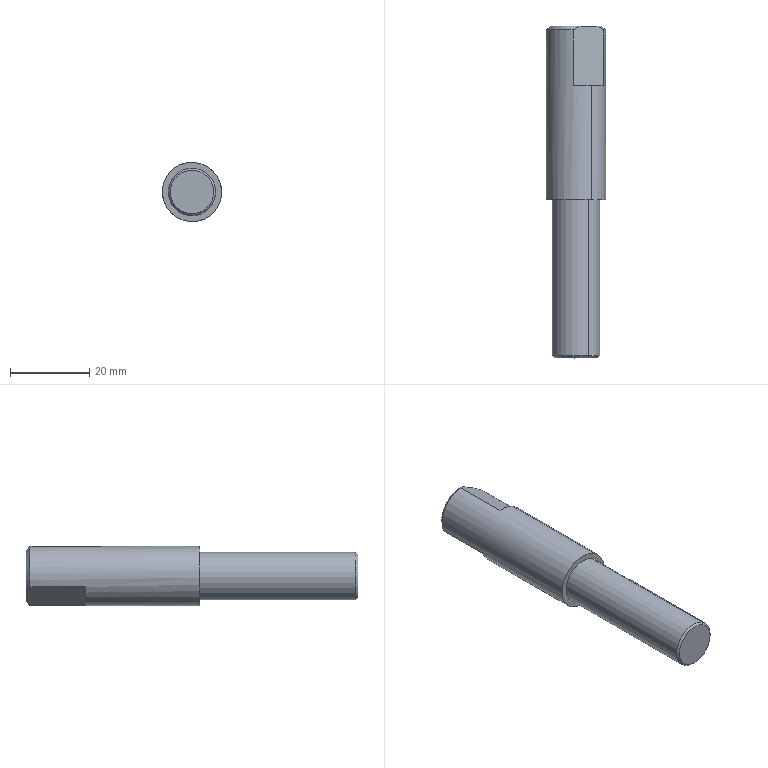Component | SolidWorks | GbgbLowerMagnetPushRodF8-1 | 1 solid | 19 faces | box 15 x 84 x 15 mm | volume 11648 mm3 | plane 7 | cone 6 | cylinder 6 | commonest cylinder face diameters 6 x2 12 x2 15 x2
build123d program:
from build123d import *

# Parameters (mm, degrees)
M6_TAPPED_HOLE1_D     = 6
M6_TAPPED_HOLE1_DEPTH = 12
M6_TAPPED_HOLE1_TIP   = 1.803
SKETCH4_OUTSIDE_W     = 34.328
SKETCH4_OUTSIDE_H     = 34.328
SKETCH4_OUTSIDE_W_2   = 23.531
SKETCH4_OUTSIDE_H_2   = 12
CUT_EXTRUDE1_DEPTH    = 15
CHAMFER2_SIZE         = 0.5
CHAMFER3_SIZE         = 1


with BuildPart() as part:
    # Sketch1 → Revolve1 (revolve)
    with BuildSketch(Plane.XY, mode=Mode.PRIVATE) as revolve1_sk:
        Polygon((0, 40), (-6, 40), (-6, 0), (-7.5, 0), (-7.5, -44), (0, -44), align=None)
    revolve(revolve1_sk.sketch.rotate(Axis((0, 59.694, 0), (0, -1, 0)), 270), axis=Axis((0, 59.694, 0), (0, -1, 0)))

    # M6 Tapped Hole1
    with Locations(Plane(origin=(0, -44, 0), x_dir=(-1, 0, 0), z_dir=(0, -1, 0))):
        with Locations((0, 0)):
            Hole(M6_TAPPED_HOLE1_D / 2, depth=M6_TAPPED_HOLE1_DEPTH)
            with Locations((0, 0, -(M6_TAPPED_HOLE1_DEPTH + M6_TAPPED_HOLE1_TIP / 2))):  # 118° drill point
                Cone(0, M6_TAPPED_HOLE1_D / 2, M6_TAPPED_HOLE1_TIP, mode=Mode.SUBTRACT)

    # Sketch4 outside → Cut-Extrude1 (cut)
    with BuildSketch(Plane.XZ.offset(44)):
        Rectangle(SKETCH4_OUTSIDE_W, SKETCH4_OUTSIDE_H)
        Rectangle(SKETCH4_OUTSIDE_W_2, SKETCH4_OUTSIDE_H_2, mode=Mode.SUBTRACT)
    extrude(amount=-CUT_EXTRUDE1_DEPTH, mode=Mode.SUBTRACT)

    # Chamfer2
    chamfer2_edges = [part.edges().sort_by_distance(p)[0] for p in [
        (0, 40, -6),
    ]]
    chamfer(chamfer2_edges, length=CHAMFER2_SIZE)

    # Chamfer3
    chamfer3_edges = [part.edges().sort_by_distance(p)[0] for p in [
        (-7.5, -44, 0),
        (7.5, -44, 0),
    ]]
    chamfer(chamfer3_edges, length=CHAMFER3_SIZE)


solid = part.part

# Placed as in the assembly
solid = solid.moved(Location((80.446, 428.93, 430.232), (0, 31.476, -180)))
STEP:
#1=CARTESIAN_POINT('',(3.054,15.312,16.754));
#2=VERTEX_POINT('',#1);
#3=CARTESIAN_POINT('',(3.28,15.312,17.123));
#4=VERTEX_POINT('',#3);
#5=CARTESIAN_POINT('',(3.167,15.312,16.938));
#6=DIRECTION('',(-0.,-1.,-0.));
#7=DIRECTION('',(-0.5221,0.,-0.8529));
#8=AXIS2_PLACEMENT_3D('',#5,#6,#7);
#9=CIRCLE('',#8,0.2165);
#10=EDGE_CURVE('',#2,#4,#9,.T.);
#11=ORIENTED_EDGE('',*,*,#10,.F.);
#12=CARTESIAN_POINT('',(3.044,15.332,16.737));
#13=VERTEX_POINT('',#12);
#14=CARTESIAN_POINT('',(3.054,15.312,16.754));
#15=DIRECTION('',(-0.3692,0.7071,-0.6031));
#16=VECTOR('',#15,39.37);
#17=LINE('',#14,#16);
#18=EDGE_CURVE('',#2,#13,#17,.T.);
#19=ORIENTED_EDGE('',*,*,#18,.T.);
#20=CARTESIAN_POINT('',(3.291,15.332,17.14));
#21=VERTEX_POINT('',#20);
#22=CARTESIAN_POINT('',(3.167,15.332,16.938));
#23=DIRECTION('',(0.,1.,0.));
#24=DIRECTION('',(-0.5221,0.,-0.8529));
#25=AXIS2_PLACEMENT_3D('',#22,#23,#24);
#26=CIRCLE('',#25,0.2362);
#27=EDGE_CURVE('',#21,#13,#26,.T.);
#28=ORIENTED_EDGE('',*,*,#27,.F.);
#29=CARTESIAN_POINT('',(3.28,15.312,17.123));
#30=DIRECTION('',(0.3692,0.7071,0.6031));
#31=VECTOR('',#30,39.37);
#32=LINE('',#29,#31);
#33=EDGE_CURVE('',#4,#21,#32,.T.);
#34=ORIENTED_EDGE('',*,*,#33,.F.);
#35=EDGE_LOOP('',(#11,#19,#28,#34));
#36=FACE_OUTER_BOUND('',#35,.T.);
#37=CARTESIAN_POINT('',(3.167,15.312,16.938));
#38=DIRECTION('',(0.,1.,0.));
#39=DIRECTION('',(0.5221,0.,0.8529));
#40=AXIS2_PLACEMENT_3D('',#37,#38,#39);
#41=CONICAL_SURFACE('',#40,0.2165,0.7854);
#42=ADVANCED_FACE('',(#36),#41,.T.);
#43=CARTESIAN_POINT('',(3.106,18.147,16.838));
#44=VERTEX_POINT('',#43);
#45=CARTESIAN_POINT('',(3.229,18.147,17.039));
#46=VERTEX_POINT('',#45);
#47=CARTESIAN_POINT('',(3.167,18.147,16.938));
#48=DIRECTION('',(0.,1.,0.));
#49=DIRECTION('',(0.5221,0.,0.8529));
#50=AXIS2_PLACEMENT_3D('',#47,#48,#49);
#51=CIRCLE('',#50,0.1181);
#52=EDGE_CURVE('',#44,#46,#51,.T.);
#53=ORIENTED_EDGE('',*,*,#52,.F.);
#54=CARTESIAN_POINT('',(3.106,18.619,16.838));
#55=VERTEX_POINT('',#54);
#56=CARTESIAN_POINT('',(3.106,18.619,16.838));
#57=DIRECTION('',(0.,1.,0.));
#58=VECTOR('',#57,39.37);
#59=LINE('',#56,#58);
#60=EDGE_CURVE('',#44,#55,#59,.T.);
#61=ORIENTED_EDGE('',*,*,#60,.T.);
#62=CARTESIAN_POINT('',(3.229,18.619,17.039));
#63=VERTEX_POINT('',#62);
#64=CARTESIAN_POINT('',(3.167,18.619,16.938));
#65=DIRECTION('',(0.,1.,0.));
#66=DIRECTION('',(0.5221,0.,0.8529));
#67=AXIS2_PLACEMENT_3D('',#64,#65,#66);
#68=CIRCLE('',#67,0.1181);
#69=EDGE_CURVE('',#55,#63,#68,.T.);
#70=ORIENTED_EDGE('',*,*,#69,.T.);
#71=CARTESIAN_POINT('',(3.229,18.619,17.039));
#72=DIRECTION('',(0.,1.,0.));
#73=VECTOR('',#72,39.37);
#74=LINE('',#71,#73);
#75=EDGE_CURVE('',#46,#63,#74,.T.);
#76=ORIENTED_EDGE('',*,*,#75,.F.);
#77=EDGE_LOOP('',(#53,#61,#70,#76));
#78=FACE_OUTER_BOUND('',#77,.T.);
#79=CARTESIAN_POINT('',(3.167,18.619,16.938));
#80=DIRECTION('',(0.,1.,0.));
#81=DIRECTION('',(0.5221,0.,0.8529));
#82=AXIS2_PLACEMENT_3D('',#79,#80,#81);
#83=CYLINDRICAL_SURFACE('',#82,0.1181);
#84=ADVANCED_FACE('',(#78),#83,.F.);
#85=CARTESIAN_POINT('',(3.167,18.076,16.938));
#86=VERTEX_POINT('',#85);
#87=CARTESIAN_POINT('',(3.229,18.147,17.039));
#88=DIRECTION('',(0.4476,0.515,0.731));
#89=VECTOR('',#88,39.37);
#90=LINE('',#87,#89);
#91=EDGE_CURVE('',#86,#46,#90,.T.);
#92=ORIENTED_EDGE('',*,*,#91,.F.);
#93=CARTESIAN_POINT('',(3.106,18.147,16.838));
#94=DIRECTION('',(-0.4476,0.515,-0.731));
#95=VECTOR('',#94,39.37);
#96=LINE('',#93,#95);
#97=EDGE_CURVE('',#86,#44,#96,.T.);
#98=ORIENTED_EDGE('',*,*,#97,.T.);
#99=ORIENTED_EDGE('',*,*,#52,.T.);
#100=EDGE_LOOP('',(#92,#98,#99));
#101=FACE_OUTER_BOUND('',#100,.T.);
#102=CARTESIAN_POINT('',(3.167,18.147,16.938));
#103=DIRECTION('',(0.,1.,0.));
#104=DIRECTION('',(0.5221,0.,0.8529));
#105=AXIS2_PLACEMENT_3D('',#102,#103,#104);
#106=CONICAL_SURFACE('',#105,0.1181,1.03);
#107=ADVANCED_FACE('',(#101),#106,.F.);
#108=CARTESIAN_POINT('',(3.044,16.887,16.737));
#109=VERTEX_POINT('',#108);
#110=CARTESIAN_POINT('',(3.291,16.887,17.14));
#111=VERTEX_POINT('',#110);
#112=CARTESIAN_POINT('',(3.167,16.887,16.938));
#113=DIRECTION('',(-0.,-1.,-0.));
#114=DIRECTION('',(-0.5221,0.,-0.8529));
#115=AXIS2_PLACEMENT_3D('',#112,#113,#114);
#116=CIRCLE('',#115,0.2362);
#117=EDGE_CURVE('',#109,#111,#116,.T.);
#118=ORIENTED_EDGE('',*,*,#117,.T.);
#119=CARTESIAN_POINT('',(3.291,14.537,17.14));
#120=DIRECTION('',(-0.,-1.,-0.));
#121=VECTOR('',#120,39.37);
#122=LINE('',#119,#121);
#123=EDGE_CURVE('',#111,#21,#122,.T.);
#124=ORIENTED_EDGE('',*,*,#123,.T.);
#125=ORIENTED_EDGE('',*,*,#27,.T.);
#126=CARTESIAN_POINT('',(3.044,14.537,16.737));
#127=DIRECTION('',(-0.,-1.,-0.));
#128=VECTOR('',#127,39.37);
#129=LINE('',#126,#128);
#130=EDGE_CURVE('',#109,#13,#129,.T.);
#131=ORIENTED_EDGE('',*,*,#130,.F.);
#132=EDGE_LOOP('',(#118,#124,#125,#131));
#133=FACE_OUTER_BOUND('',#132,.T.);
#134=CARTESIAN_POINT('',(3.167,14.537,16.938));
#135=DIRECTION('',(-0.,-1.,-0.));
#136=DIRECTION('',(-0.5221,0.,-0.8529));
#137=AXIS2_PLACEMENT_3D('',#134,#135,#136);
#138=CYLINDRICAL_SURFACE('',#137,0.2362);
#139=ADVANCED_FACE('',(#133),#138,.T.);
#140=CARTESIAN_POINT('',(3.442,18.029,17.047));
#141=VERTEX_POINT('',#140);
#142=CARTESIAN_POINT('',(3.321,18.029,17.19));
#143=VERTEX_POINT('',#142);
#144=CARTESIAN_POINT('',(3.167,18.029,16.938));
#145=DIRECTION('',(-0.,-1.,-0.));
#146=DIRECTION('',(0.5221,0.,0.8529));
#147=AXIS2_PLACEMENT_3D('',#144,#145,#146);
#148=CIRCLE('',#147,0.2953);
#149=EDGE_CURVE('',#141,#143,#148,.T.);
#150=ORIENTED_EDGE('',*,*,#149,.T.);
#151=CARTESIAN_POINT('',(3.321,16.887,17.19));
#152=VERTEX_POINT('',#151);
#153=CARTESIAN_POINT('',(3.321,14.537,17.19));
#154=DIRECTION('',(-0.,-1.,-0.));
#155=VECTOR('',#154,39.37);
#156=LINE('',#153,#155);
#157=EDGE_CURVE('',#143,#152,#156,.T.);
#158=ORIENTED_EDGE('',*,*,#157,.T.);
#159=CARTESIAN_POINT('',(3.013,16.887,16.686));
#160=VERTEX_POINT('',#159);
#161=CARTESIAN_POINT('',(3.167,16.887,16.938));
#162=DIRECTION('',(-0.,-1.,-0.));
#163=DIRECTION('',(-0.5221,0.,-0.8529));
#164=AXIS2_PLACEMENT_3D('',#161,#162,#163);
#165=CIRCLE('',#164,0.2953);
#166=EDGE_CURVE('',#160,#152,#165,.T.);
#167=ORIENTED_EDGE('',*,*,#166,.F.);
#168=CARTESIAN_POINT('',(3.013,18.029,16.686));
#169=VERTEX_POINT('',#168);
#170=CARTESIAN_POINT('',(3.013,14.537,16.686));
#171=DIRECTION('',(-0.,-1.,-0.));
#172=VECTOR('',#171,39.37);
#173=LINE('',#170,#172);
#174=EDGE_CURVE('',#169,#160,#173,.T.);
#175=ORIENTED_EDGE('',*,*,#174,.F.);
#176=CARTESIAN_POINT('',(3.195,18.029,16.644));
#177=VERTEX_POINT('',#176);
#178=CARTESIAN_POINT('',(3.167,18.029,16.938));
#179=DIRECTION('',(-0.,-1.,-0.));
#180=DIRECTION('',(0.5221,0.,0.8529));
#181=AXIS2_PLACEMENT_3D('',#178,#179,#180);
#182=CIRCLE('',#181,0.2953);
#183=EDGE_CURVE('',#169,#177,#182,.T.);
#184=ORIENTED_EDGE('',*,*,#183,.T.);
#185=CARTESIAN_POINT('',(3.195,18.58,16.644));
#186=VERTEX_POINT('',#185);
#187=CARTESIAN_POINT('',(3.195,14.537,16.644));
#188=DIRECTION('',(0.,1.,0.));
#189=VECTOR('',#188,39.37);
#190=LINE('',#187,#189);
#191=EDGE_CURVE('',#177,#186,#190,.T.);
#192=ORIENTED_EDGE('',*,*,#191,.T.);
#193=CARTESIAN_POINT('',(3.442,18.58,17.047));
#194=VERTEX_POINT('',#193);
#195=CARTESIAN_POINT('',(3.167,18.58,16.938));
#196=DIRECTION('',(-0.,-1.,-0.));
#197=DIRECTION('',(0.5221,0.,0.8529));
#198=AXIS2_PLACEMENT_3D('',#195,#196,#197);
#199=CIRCLE('',#198,0.2953);
#200=EDGE_CURVE('',#186,#194,#199,.T.);
#201=ORIENTED_EDGE('',*,*,#200,.T.);
#202=CARTESIAN_POINT('',(3.442,14.537,17.047));
#203=DIRECTION('',(-0.,-1.,-0.));
#204=VECTOR('',#203,39.37);
#205=LINE('',#202,#204);
#206=EDGE_CURVE('',#194,#141,#205,.T.);
#207=ORIENTED_EDGE('',*,*,#206,.T.);
#208=EDGE_LOOP('',(#150,#158,#167,#175,#184,#192,#201,#207));
#209=FACE_OUTER_BOUND('',#208,.T.);
#210=CARTESIAN_POINT('',(3.167,14.537,16.938));
#211=DIRECTION('',(-0.,-1.,-0.));
#212=DIRECTION('',(-0.5221,0.,-0.8529));
#213=AXIS2_PLACEMENT_3D('',#210,#211,#212);
#214=CYLINDRICAL_SURFACE('',#213,0.2953);
#215=ADVANCED_FACE('',(#209),#214,.T.);
#216=ORIENTED_EDGE('',*,*,#157,.F.);
#217=CARTESIAN_POINT('',(3.139,18.029,17.232));
#218=VERTEX_POINT('',#217);
#219=CARTESIAN_POINT('',(3.167,18.029,16.938));
#220=DIRECTION('',(-0.,-1.,-0.));
#221=DIRECTION('',(0.5221,0.,0.8529));
#222=AXIS2_PLACEMENT_3D('',#219,#220,#221);
#223=CIRCLE('',#222,0.2953);
#224=EDGE_CURVE('',#143,#218,#223,.T.);
#225=ORIENTED_EDGE('',*,*,#224,.T.);
#226=CARTESIAN_POINT('',(3.139,18.58,17.232));
#227=VERTEX_POINT('',#226);
#228=CARTESIAN_POINT('',(3.139,14.537,17.232));
#229=DIRECTION('',(0.,1.,0.));
#230=VECTOR('',#229,39.37);
#231=LINE('',#228,#230);
#232=EDGE_CURVE('',#218,#227,#231,.T.);
#233=ORIENTED_EDGE('',*,*,#232,.T.);
#234=CARTESIAN_POINT('',(2.893,18.58,16.829));
#235=VERTEX_POINT('',#234);
#236=CARTESIAN_POINT('',(3.167,18.58,16.938));
#237=DIRECTION('',(-0.,-1.,-0.));
#238=DIRECTION('',(0.5221,0.,0.8529));
#239=AXIS2_PLACEMENT_3D('',#236,#237,#238);
#240=CIRCLE('',#239,0.2953);
#241=EDGE_CURVE('',#227,#235,#240,.T.);
#242=ORIENTED_EDGE('',*,*,#241,.T.);
#243=CARTESIAN_POINT('',(2.893,18.029,16.829));
#244=VERTEX_POINT('',#243);
#245=CARTESIAN_POINT('',(2.893,14.537,16.829));
#246=DIRECTION('',(-0.,-1.,-0.));
#247=VECTOR('',#246,39.37);
#248=LINE('',#245,#247);
#249=EDGE_CURVE('',#235,#244,#248,.T.);
#250=ORIENTED_EDGE('',*,*,#249,.T.);
#251=CARTESIAN_POINT('',(3.167,18.029,16.938));
#252=DIRECTION('',(-0.,-1.,-0.));
#253=DIRECTION('',(0.5221,0.,0.8529));
#254=AXIS2_PLACEMENT_3D('',#251,#252,#253);
#255=CIRCLE('',#254,0.2953);
#256=EDGE_CURVE('',#244,#169,#255,.T.);
#257=ORIENTED_EDGE('',*,*,#256,.T.);
#258=ORIENTED_EDGE('',*,*,#174,.T.);
#259=CARTESIAN_POINT('',(3.167,16.887,16.938));
#260=DIRECTION('',(-0.,-1.,-0.));
#261=DIRECTION('',(-0.5221,0.,-0.8529));
#262=AXIS2_PLACEMENT_3D('',#259,#260,#261);
#263=CIRCLE('',#262,0.2953);
#264=EDGE_CURVE('',#152,#160,#263,.T.);
#265=ORIENTED_EDGE('',*,*,#264,.F.);
#266=EDGE_LOOP('',(#216,#225,#233,#242,#250,#257,#258,#265));
#267=FACE_OUTER_BOUND('',#266,.T.);
#268=CARTESIAN_POINT('',(3.167,14.537,16.938));
#269=DIRECTION('',(-0.,-1.,-0.));
#270=DIRECTION('',(-0.5221,0.,-0.8529));
#271=AXIS2_PLACEMENT_3D('',#268,#269,#270);
#272=CYLINDRICAL_SURFACE('',#271,0.2953);
#273=ADVANCED_FACE('',(#267),#272,.T.);
#274=CARTESIAN_POINT('',(3.167,18.619,16.938));
#275=DIRECTION('',(0.,1.,0.));
#276=DIRECTION('',(0.5221,0.,0.8529));
#277=AXIS2_PLACEMENT_3D('',#274,#275,#276);
#278=CIRCLE('',#277,0.1181);
#279=EDGE_CURVE('',#63,#55,#278,.T.);
#280=ORIENTED_EDGE('',*,*,#279,.F.);
#281=ORIENTED_EDGE('',*,*,#69,.F.);
#282=EDGE_LOOP('',(#280,#281));
#283=FACE_BOUND('',#282,.T.);
#284=CARTESIAN_POINT('',(3.207,18.619,17.191));
#285=VERTEX_POINT('',#284);
#286=CARTESIAN_POINT('',(3.374,18.619,17.088));
#287=VERTEX_POINT('',#286);
#288=CARTESIAN_POINT('',(3.039,18.619,17.294));
#289=DIRECTION('',(0.8529,-0.,-0.5221));
#290=VECTOR('',#289,39.37);
#291=LINE('',#288,#290);
#292=EDGE_CURVE('',#285,#287,#291,.T.);
#293=ORIENTED_EDGE('',*,*,#292,.T.);
#294=CARTESIAN_POINT('',(3.128,18.619,16.685));
#295=VERTEX_POINT('',#294);
#296=CARTESIAN_POINT('',(3.167,18.619,16.938));
#297=DIRECTION('',(0.,1.,0.));
#298=DIRECTION('',(0.5221,0.,0.8529));
#299=AXIS2_PLACEMENT_3D('',#296,#297,#298);
#300=CIRCLE('',#299,0.2559);
#301=EDGE_CURVE('',#287,#295,#300,.T.);
#302=ORIENTED_EDGE('',*,*,#301,.T.);
#303=CARTESIAN_POINT('',(2.96,18.619,16.788));
#304=VERTEX_POINT('',#303);
#305=CARTESIAN_POINT('',(2.792,18.619,16.891));
#306=DIRECTION('',(-0.8529,0.,0.5221));
#307=VECTOR('',#306,39.37);
#308=LINE('',#305,#307);
#309=EDGE_CURVE('',#295,#304,#308,.T.);
#310=ORIENTED_EDGE('',*,*,#309,.T.);
#311=CARTESIAN_POINT('',(3.167,18.619,16.938));
#312=DIRECTION('',(0.,1.,0.));
#313=DIRECTION('',(0.5221,0.,0.8529));
#314=AXIS2_PLACEMENT_3D('',#311,#312,#313);
#315=CIRCLE('',#314,0.2559);
#316=EDGE_CURVE('',#304,#285,#315,.T.);
#317=ORIENTED_EDGE('',*,*,#316,.T.);
#318=EDGE_LOOP('',(#293,#302,#310,#317));
#319=FACE_OUTER_BOUND('',#318,.T.);
#320=CARTESIAN_POINT('',(2.915,18.619,17.092));
#321=DIRECTION('',(0.,1.,0.));
#322=DIRECTION('',(0.5221,-0.,0.8529));
#323=AXIS2_PLACEMENT_3D('',#320,#321,#322);
#324=PLANE('',#323);
#325=ADVANCED_FACE('',(#283,#319),#324,.T.);
#326=CARTESIAN_POINT('',(3.167,15.312,16.938));
#327=DIRECTION('',(-0.,-1.,-0.));
#328=DIRECTION('',(-0.5221,0.,-0.8529));
#329=AXIS2_PLACEMENT_3D('',#326,#327,#328);
#330=CIRCLE('',#329,0.2165);
#331=EDGE_CURVE('',#4,#2,#330,.T.);
#332=ORIENTED_EDGE('',*,*,#331,.T.);
#333=ORIENTED_EDGE('',*,*,#10,.T.);
#334=EDGE_LOOP('',(#332,#333));
#335=FACE_OUTER_BOUND('',#334,.T.);
#336=CARTESIAN_POINT('',(3.167,15.312,16.938));
#337=DIRECTION('',(-0.,-1.,-0.));
#338=DIRECTION('',(-0.5221,0.,-0.8529));
#339=AXIS2_PLACEMENT_3D('',#336,#337,#338);
#340=PLANE('',#339);
#341=ADVANCED_FACE('',(#335),#340,.T.);
#342=ORIENTED_EDGE('',*,*,#123,.F.);
#343=CARTESIAN_POINT('',(3.167,16.887,16.938));
#344=DIRECTION('',(-0.,-1.,-0.));
#345=DIRECTION('',(-0.5221,0.,-0.8529));
#346=AXIS2_PLACEMENT_3D('',#343,#344,#345);
#347=CIRCLE('',#346,0.2362);
#348=EDGE_CURVE('',#111,#109,#347,.T.);
#349=ORIENTED_EDGE('',*,*,#348,.T.);
#350=ORIENTED_EDGE('',*,*,#130,.T.);
#351=CARTESIAN_POINT('',(3.167,15.332,16.938));
#352=DIRECTION('',(0.,1.,0.));
#353=DIRECTION('',(-0.5221,0.,-0.8529));
#354=AXIS2_PLACEMENT_3D('',#351,#352,#353);
#355=CIRCLE('',#354,0.2362);
#356=EDGE_CURVE('',#13,#21,#355,.T.);
#357=ORIENTED_EDGE('',*,*,#356,.T.);
#358=EDGE_LOOP('',(#342,#349,#350,#357));
#359=FACE_OUTER_BOUND('',#358,.T.);
#360=CARTESIAN_POINT('',(3.167,14.537,16.938));
#361=DIRECTION('',(-0.,-1.,-0.));
#362=DIRECTION('',(-0.5221,0.,-0.8529));
#363=AXIS2_PLACEMENT_3D('',#360,#361,#362);
#364=CYLINDRICAL_SURFACE('',#363,0.2362);
#365=ADVANCED_FACE('',(#359),#364,.T.);
#366=ORIENTED_EDGE('',*,*,#166,.T.);
#367=ORIENTED_EDGE('',*,*,#264,.T.);
#368=EDGE_LOOP('',(#366,#367));
#369=FACE_OUTER_BOUND('',#368,.T.);
#370=ORIENTED_EDGE('',*,*,#117,.F.);
#371=ORIENTED_EDGE('',*,*,#348,.F.);
#372=EDGE_LOOP('',(#370,#371));
#373=FACE_BOUND('',#372,.T.);
#374=CARTESIAN_POINT('',(2.966,16.887,17.062));
#375=DIRECTION('',(-0.,-1.,-0.));
#376=DIRECTION('',(-0.5221,0.,-0.8529));
#377=AXIS2_PLACEMENT_3D('',#374,#375,#376);
#378=PLANE('',#377);
#379=ADVANCED_FACE('',(#369,#373),#378,.T.);
#380=ORIENTED_EDGE('',*,*,#97,.F.);
#381=ORIENTED_EDGE('',*,*,#91,.T.);
#382=CARTESIAN_POINT('',(3.167,18.147,16.938));
#383=DIRECTION('',(0.,1.,0.));
#384=DIRECTION('',(0.5221,0.,0.8529));
#385=AXIS2_PLACEMENT_3D('',#382,#383,#384);
#386=CIRCLE('',#385,0.1181);
#387=EDGE_CURVE('',#46,#44,#386,.T.);
#388=ORIENTED_EDGE('',*,*,#387,.T.);
#389=EDGE_LOOP('',(#380,#381,#388));
#390=FACE_OUTER_BOUND('',#389,.T.);
#391=CARTESIAN_POINT('',(3.167,18.147,16.938));
#392=DIRECTION('',(0.,1.,0.));
#393=DIRECTION('',(0.5221,0.,0.8529));
#394=AXIS2_PLACEMENT_3D('',#391,#392,#393);
#395=CONICAL_SURFACE('',#394,0.1181,1.03);
#396=ADVANCED_FACE('',(#390),#395,.F.);
#397=ORIENTED_EDGE('',*,*,#60,.F.);
#398=ORIENTED_EDGE('',*,*,#387,.F.);
#399=ORIENTED_EDGE('',*,*,#75,.T.);
#400=ORIENTED_EDGE('',*,*,#279,.T.);
#401=EDGE_LOOP('',(#397,#398,#399,#400));
#402=FACE_OUTER_BOUND('',#401,.T.);
#403=CARTESIAN_POINT('',(3.167,18.619,16.938));
#404=DIRECTION('',(0.,1.,0.));
#405=DIRECTION('',(0.5221,0.,0.8529));
#406=AXIS2_PLACEMENT_3D('',#403,#404,#405);
#407=CYLINDRICAL_SURFACE('',#406,0.1181);
#408=ADVANCED_FACE('',(#402),#407,.F.);
#409=ORIENTED_EDGE('',*,*,#309,.F.);
#410=CARTESIAN_POINT('',(3.128,18.619,16.685));
#411=CARTESIAN_POINT('',(3.151,18.609,16.671));
#412=CARTESIAN_POINT('',(3.173,18.595,16.657));
#413=CARTESIAN_POINT('',(3.195,18.58,16.644));
#414=B_SPLINE_CURVE_WITH_KNOTS('',3,(#410,#411,#412,#413),.UNSPECIFIED.,.F.,.F.,(4,4),(0.,0.002236),.UNSPECIFIED.);
#415=EDGE_CURVE('',#295,#186,#414,.T.);
#416=ORIENTED_EDGE('',*,*,#415,.T.);
#417=ORIENTED_EDGE('',*,*,#191,.F.);
#418=CARTESIAN_POINT('',(2.649,18.029,16.979));
#419=DIRECTION('',(-0.8529,0.,0.5221));
#420=VECTOR('',#419,39.37);
#421=LINE('',#418,#420);
#422=EDGE_CURVE('',#177,#244,#421,.T.);
#423=ORIENTED_EDGE('',*,*,#422,.T.);
#424=ORIENTED_EDGE('',*,*,#249,.F.);
#425=CARTESIAN_POINT('',(2.893,18.58,16.829));
#426=CARTESIAN_POINT('',(2.914,18.595,16.816));
#427=CARTESIAN_POINT('',(2.936,18.609,16.803));
#428=CARTESIAN_POINT('',(2.96,18.619,16.788));
#429=B_SPLINE_CURVE_WITH_KNOTS('',3,(#425,#426,#427,#428),.UNSPECIFIED.,.F.,.F.,(4,4),(0.,0.002236),.UNSPECIFIED.);
#430=EDGE_CURVE('',#235,#304,#429,.T.);
#431=ORIENTED_EDGE('',*,*,#430,.T.);
#432=EDGE_LOOP('',(#409,#416,#417,#423,#424,#431));
#433=FACE_OUTER_BOUND('',#432,.T.);
#434=CARTESIAN_POINT('',(2.649,18.029,16.979));
#435=DIRECTION('',(-0.5221,0.,-0.8529));
#436=DIRECTION('',(0.8529,-0.,-0.5221));
#437=AXIS2_PLACEMENT_3D('',#434,#435,#436);
#438=PLANE('',#437);
#439=ADVANCED_FACE('',(#433),#438,.T.);
#440=ORIENTED_EDGE('',*,*,#422,.F.);
#441=ORIENTED_EDGE('',*,*,#183,.F.);
#442=ORIENTED_EDGE('',*,*,#256,.F.);
#443=EDGE_LOOP('',(#440,#441,#442));
#444=FACE_OUTER_BOUND('',#443,.T.);
#445=CARTESIAN_POINT('',(3.167,18.029,16.938));
#446=DIRECTION('',(0.,1.,0.));
#447=DIRECTION('',(0.5221,-0.,0.8529));
#448=AXIS2_PLACEMENT_3D('',#445,#446,#447);
#449=PLANE('',#448);
#450=ADVANCED_FACE('',(#444),#449,.T.);
#451=CARTESIAN_POINT('',(2.895,18.029,17.382));
#452=DIRECTION('',(0.8529,-0.,-0.5221));
#453=VECTOR('',#452,39.37);
#454=LINE('',#451,#453);
#455=EDGE_CURVE('',#218,#141,#454,.T.);
#456=ORIENTED_EDGE('',*,*,#455,.F.);
#457=ORIENTED_EDGE('',*,*,#224,.F.);
#458=ORIENTED_EDGE('',*,*,#149,.F.);
#459=EDGE_LOOP('',(#456,#457,#458));
#460=FACE_OUTER_BOUND('',#459,.T.);
#461=CARTESIAN_POINT('',(3.167,18.029,16.938));
#462=DIRECTION('',(0.,1.,0.));
#463=DIRECTION('',(0.5221,-0.,0.8529));
#464=AXIS2_PLACEMENT_3D('',#461,#462,#463);
#465=PLANE('',#464);
#466=ADVANCED_FACE('',(#460),#465,.T.);
#467=ORIENTED_EDGE('',*,*,#206,.F.);
#468=CARTESIAN_POINT('',(3.442,18.58,17.047));
#469=CARTESIAN_POINT('',(3.42,18.595,17.06));
#470=CARTESIAN_POINT('',(3.398,18.609,17.074));
#471=CARTESIAN_POINT('',(3.374,18.619,17.088));
#472=B_SPLINE_CURVE_WITH_KNOTS('',3,(#468,#469,#470,#471),.UNSPECIFIED.,.F.,.F.,(4,4),(0.,0.002236),.UNSPECIFIED.);
#473=EDGE_CURVE('',#194,#287,#472,.T.);
#474=ORIENTED_EDGE('',*,*,#473,.T.);
#475=ORIENTED_EDGE('',*,*,#292,.F.);
#476=CARTESIAN_POINT('',(3.207,18.619,17.191));
#477=CARTESIAN_POINT('',(3.183,18.609,17.205));
#478=CARTESIAN_POINT('',(3.161,18.595,17.219));
#479=CARTESIAN_POINT('',(3.139,18.58,17.232));
#480=B_SPLINE_CURVE_WITH_KNOTS('',3,(#476,#477,#478,#479),.UNSPECIFIED.,.F.,.F.,(4,4),(0.,0.002236),.UNSPECIFIED.);
#481=EDGE_CURVE('',#285,#227,#480,.T.);
#482=ORIENTED_EDGE('',*,*,#481,.T.);
#483=ORIENTED_EDGE('',*,*,#232,.F.);
#484=ORIENTED_EDGE('',*,*,#455,.T.);
#485=EDGE_LOOP('',(#467,#474,#475,#482,#483,#484));
#486=FACE_OUTER_BOUND('',#485,.T.);
#487=CARTESIAN_POINT('',(2.895,18.029,17.382));
#488=DIRECTION('',(0.5221,-0.,0.8529));
#489=DIRECTION('',(-0.8529,0.,0.5221));
#490=AXIS2_PLACEMENT_3D('',#487,#488,#489);
#491=PLANE('',#490);
#492=ADVANCED_FACE('',(#486),#491,.T.);
#493=ORIENTED_EDGE('',*,*,#18,.F.);
#494=ORIENTED_EDGE('',*,*,#331,.F.);
#495=ORIENTED_EDGE('',*,*,#33,.T.);
#496=ORIENTED_EDGE('',*,*,#356,.F.);
#497=EDGE_LOOP('',(#493,#494,#495,#496));
#498=FACE_OUTER_BOUND('',#497,.T.);
#499=CARTESIAN_POINT('',(3.167,15.312,16.938));
#500=DIRECTION('',(0.,1.,0.));
#501=DIRECTION('',(0.5221,0.,0.8529));
#502=AXIS2_PLACEMENT_3D('',#499,#500,#501);
#503=CONICAL_SURFACE('',#502,0.2165,0.7854);
#504=ADVANCED_FACE('',(#498),#503,.T.);
#505=ORIENTED_EDGE('',*,*,#415,.F.);
#506=ORIENTED_EDGE('',*,*,#301,.F.);
#507=ORIENTED_EDGE('',*,*,#473,.F.);
#508=ORIENTED_EDGE('',*,*,#200,.F.);
#509=EDGE_LOOP('',(#505,#506,#507,#508));
#510=FACE_OUTER_BOUND('',#509,.T.);
#511=CARTESIAN_POINT('',(3.167,18.58,16.938));
#512=DIRECTION('',(-0.,-1.,-0.));
#513=DIRECTION('',(-0.5221,0.,-0.8529));
#514=AXIS2_PLACEMENT_3D('',#511,#512,#513);
#515=CONICAL_SURFACE('',#514,0.2953,0.7854);
#516=ADVANCED_FACE('',(#510),#515,.T.);
#517=ORIENTED_EDGE('',*,*,#481,.F.);
#518=ORIENTED_EDGE('',*,*,#316,.F.);
#519=ORIENTED_EDGE('',*,*,#430,.F.);
#520=ORIENTED_EDGE('',*,*,#241,.F.);
#521=EDGE_LOOP('',(#517,#518,#519,#520));
#522=FACE_OUTER_BOUND('',#521,.T.);
#523=CARTESIAN_POINT('',(3.167,18.58,16.938));
#524=DIRECTION('',(-0.,-1.,-0.));
#525=DIRECTION('',(-0.5221,0.,-0.8529));
#526=AXIS2_PLACEMENT_3D('',#523,#524,#525);
#527=CONICAL_SURFACE('',#526,0.2953,0.7854);
#528=ADVANCED_FACE('',(#522),#527,.T.);
#529=CLOSED_SHELL('',(#42,#84,#107,#139,#215,#273,#325,#341,#365,#379,#396,#408,#439,#450,#466,#492,#504,#516,#528));
#530=MANIFOLD_SOLID_BREP('',#529);
#531=CARTESIAN_POINT('',(0.,0.,0.));
#532=DIRECTION('',(0.,0.,1.));
#533=DIRECTION('',(1.,0.,0.));
#534=AXIS2_PLACEMENT_3D('',#531,#532,#533);
#535=(LENGTH_UNIT()NAMED_UNIT(*)SI_UNIT($,.METRE.));
#536=LENGTH_MEASURE_WITH_UNIT(LENGTH_MEASURE(0.0254),#535);
#537=DIMENSIONAL_EXPONENTS(1.,0.,0.,0.,0.,0.,0.);
#538=(CONVERSION_BASED_UNIT('',#536)LENGTH_UNIT()NAMED_UNIT(#537));
#539=UNCERTAINTY_MEASURE_WITH_UNIT(LENGTH_MEASURE(0.00001),#538,'','');
#540=(NAMED_UNIT(*)PLANE_ANGLE_UNIT()SI_UNIT($,.RADIAN.));
#541=(NAMED_UNIT(*)SI_UNIT($,.STERADIAN.)SOLID_ANGLE_UNIT());
#542=(GEOMETRIC_REPRESENTATION_CONTEXT(3)GLOBAL_UNCERTAINTY_ASSIGNED_CONTEXT((#539))GLOBAL_UNIT_ASSIGNED_CONTEXT((#538,#540,#541))REPRESENTATION_CONTEXT('',''));
#543=ADVANCED_BREP_SHAPE_REPRESENTATION('',(#530,#534),#542);
#544=COLOUR_RGB('',0.7922,0.8196,0.9333);
#545=FILL_AREA_STYLE_COLOUR('',#544);
#546=FILL_AREA_STYLE('',(#545));
#547=SURFACE_STYLE_FILL_AREA(#546);
#548=SURFACE_SIDE_STYLE('',(#547));
#549=SURFACE_STYLE_USAGE(.BOTH.,#548);
#550=PRESENTATION_STYLE_ASSIGNMENT((#549));
#551=STYLED_ITEM('',(#550),#530);
#552=(LENGTH_UNIT()NAMED_UNIT(*)SI_UNIT($,.METRE.));
#553=LENGTH_MEASURE_WITH_UNIT(LENGTH_MEASURE(0.0254),#552);
#554=DIMENSIONAL_EXPONENTS(1.,0.,0.,0.,0.,0.,0.);
#555=(CONVERSION_BASED_UNIT('',#553)LENGTH_UNIT()NAMED_UNIT(#554));
#556=UNCERTAINTY_MEASURE_WITH_UNIT(LENGTH_MEASURE(0.00001),#555,'','');
#557=(NAMED_UNIT(*)PLANE_ANGLE_UNIT()SI_UNIT($,.RADIAN.));
#558=(NAMED_UNIT(*)SI_UNIT($,.STERADIAN.)SOLID_ANGLE_UNIT());
#559=(GEOMETRIC_REPRESENTATION_CONTEXT(3)GLOBAL_UNCERTAINTY_ASSIGNED_CONTEXT((#556))GLOBAL_UNIT_ASSIGNED_CONTEXT((#555,#557,#558))REPRESENTATION_CONTEXT('',''));
#560=MECHANICAL_DESIGN_GEOMETRIC_PRESENTATION_REPRESENTATION('',(#551),#559);
#561=PRESENTATION_LAYER_ASSIGNMENT('','',(#551));